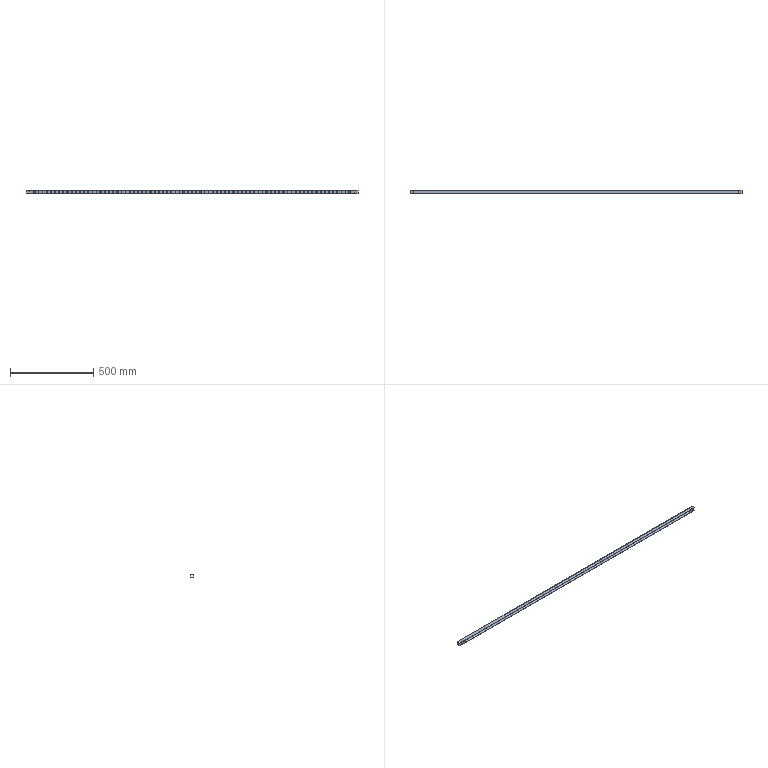Component | SolidWorks | FrontDoorAssembly-1_FrontDoorWelding-1_DoorLongitudinalStiffenerPG50-02-102-3 | 5 solids | 232 faces | volume 166218 mm3 | cylinder 158 | plane 66 | cone 8 | commonest cylinder face diameters 4.6 x110 10 x36 3.3 x6 0.3 x6 | material AISI 1045 Steel, cold drawn